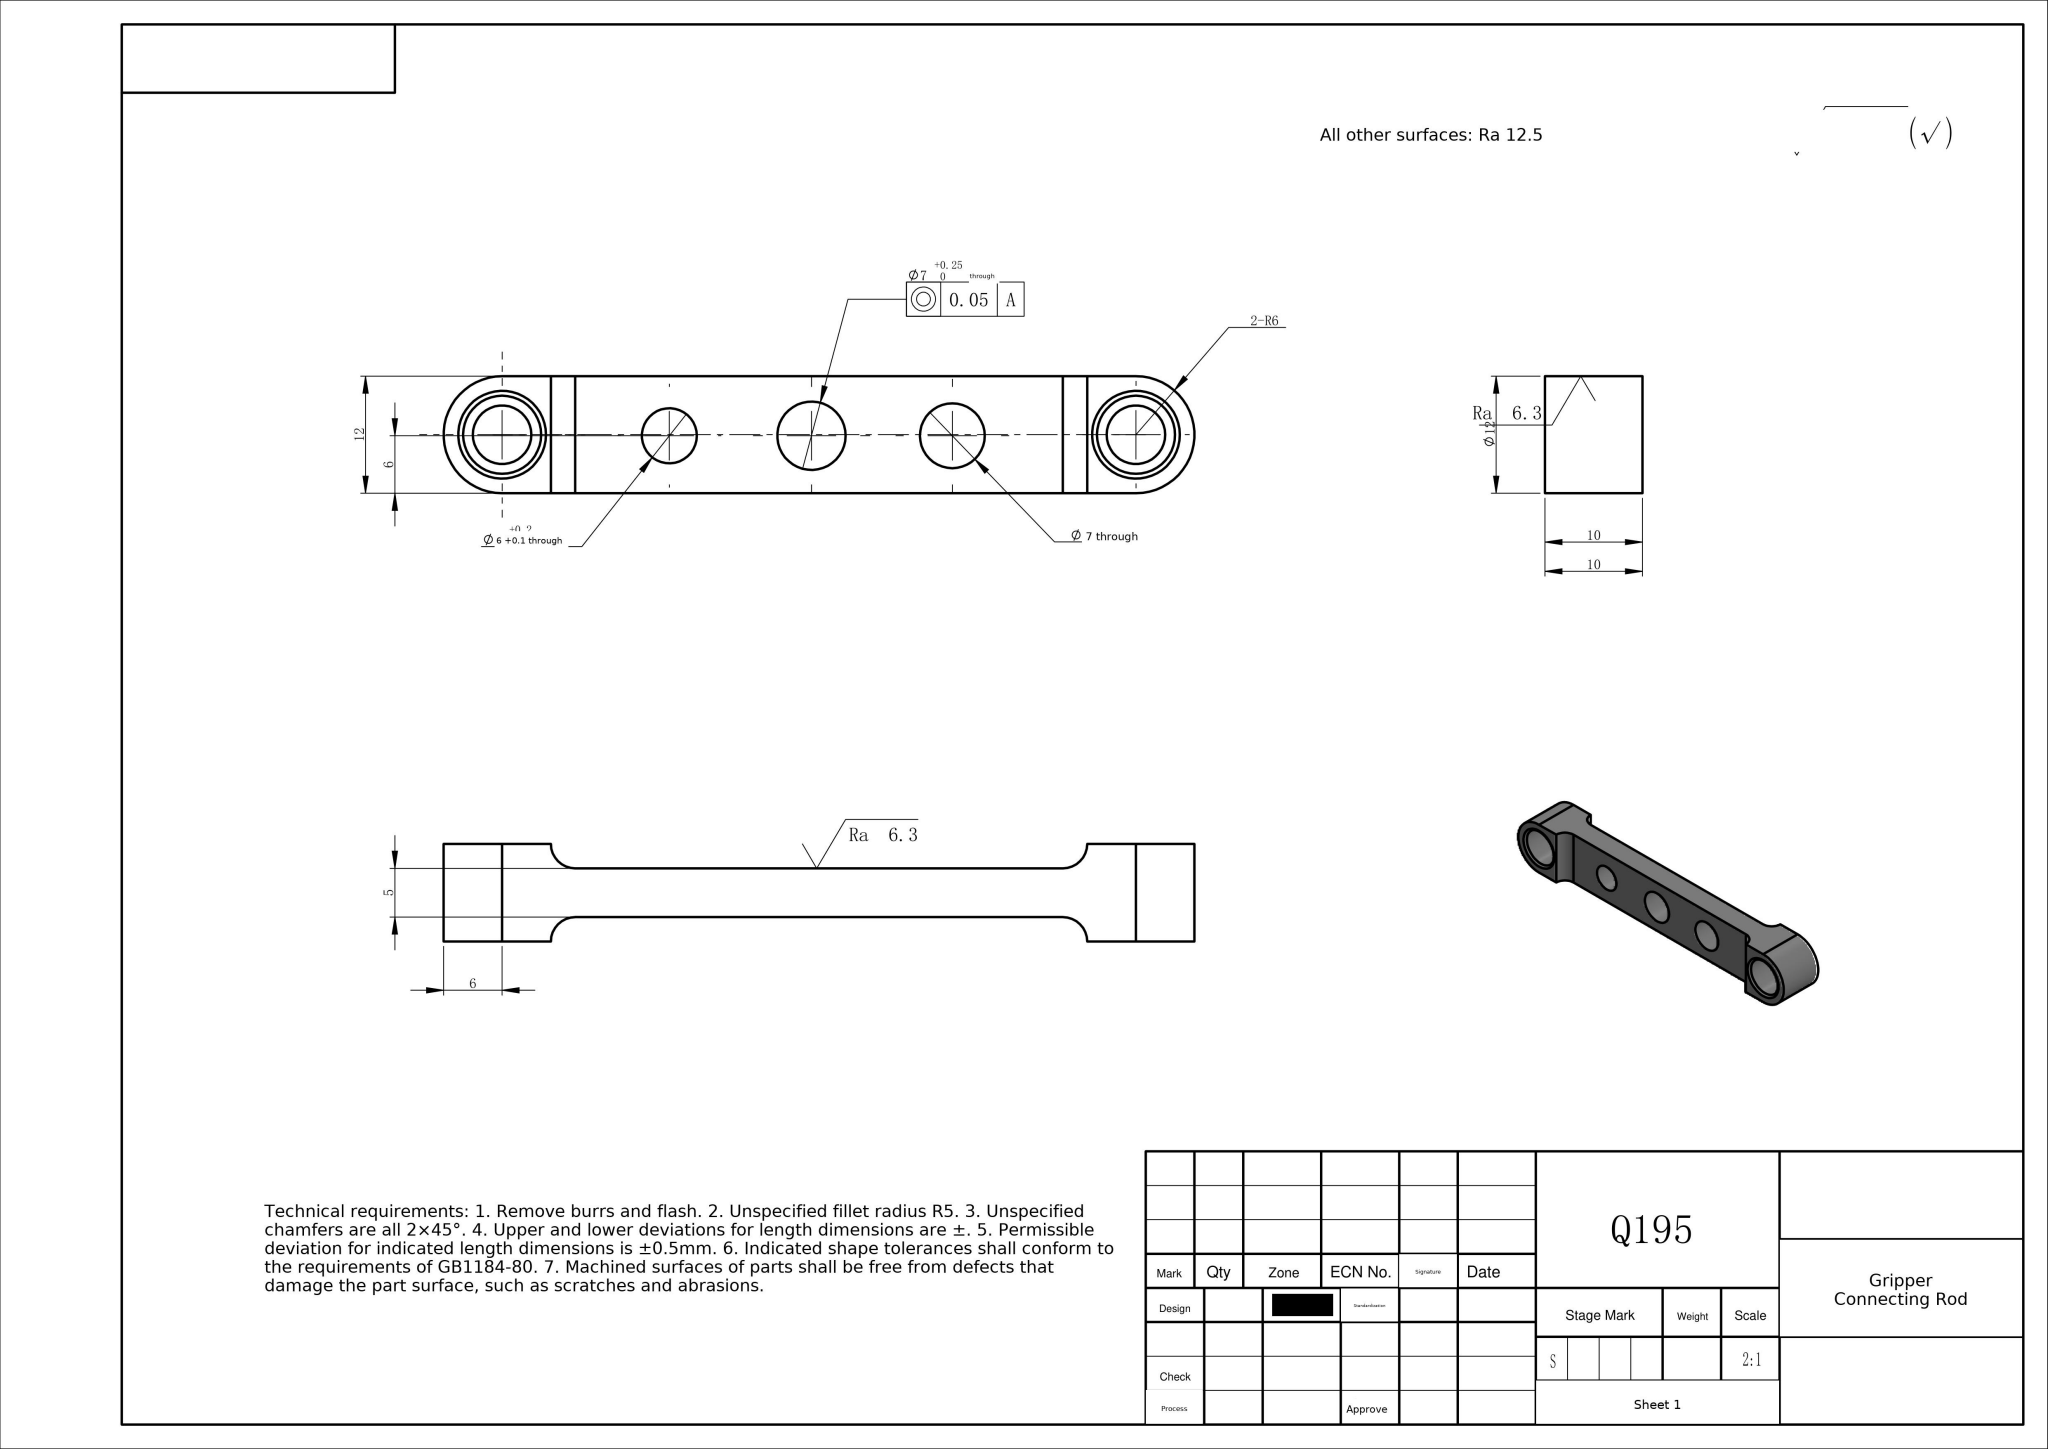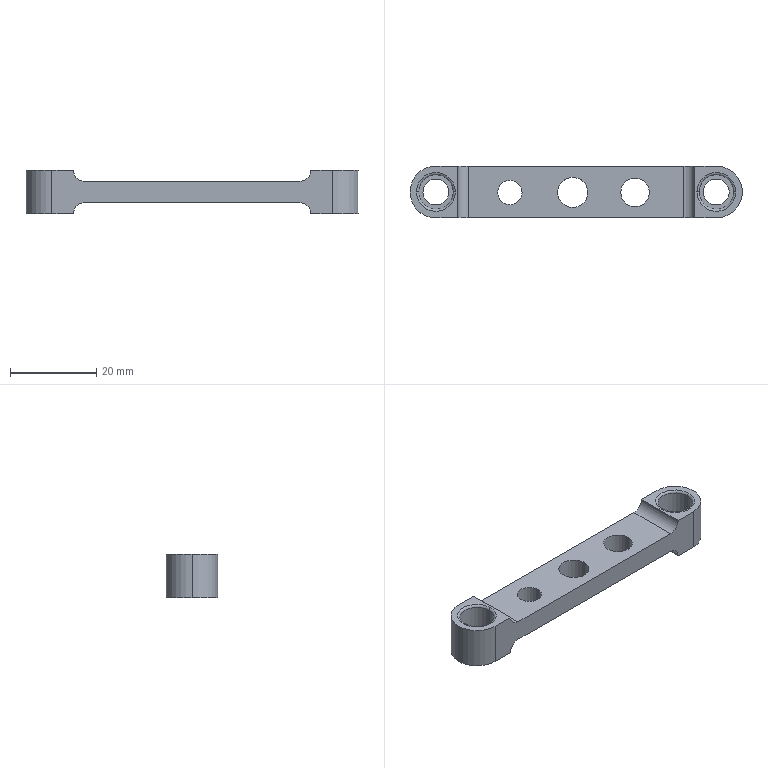Part | SolidWorks | drawing in inches | material Q195 | 1 solid | 35 faces | box 77 x 12 x 10 mm | volume 4284 mm3 | cylinder 21 | plane 10 | torus 4 | commonest cylinder face diameters 6 x4 8 x4 5 x4 12 x3 6.646 x2 7.005 x2 5.641 x2